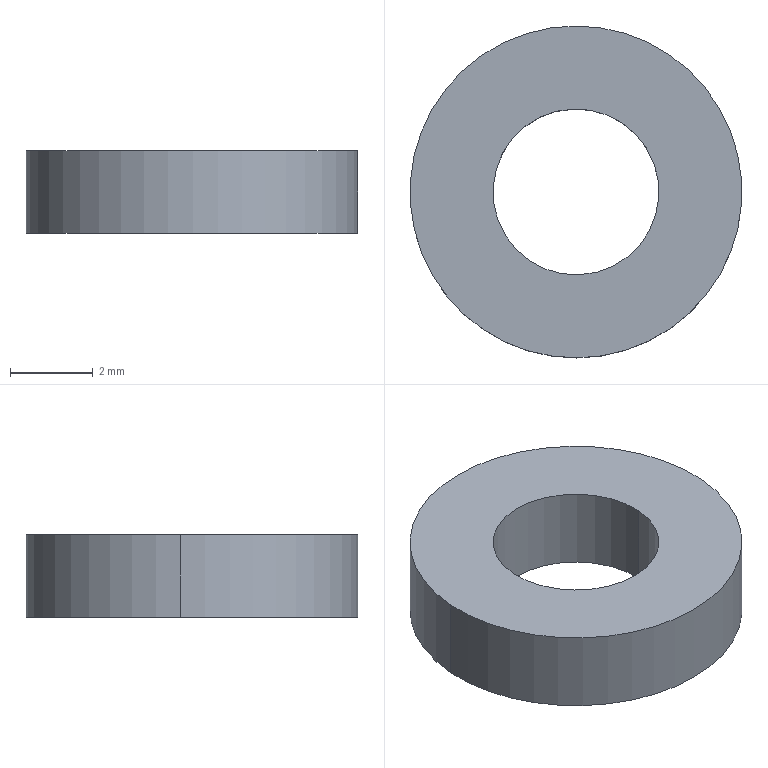Component | SolidWorks | FrontAxisWasher-3 | 1 solid | 6 faces | box 8 x 8 x 2 mm | volume 75 mm3 | cylinder 4 | plane 2 | commonest cylinder face diameters 4 x2 8 x2
build123d program:
from build123d import *

# Parameters (mm, degrees)
SKETCH1_R           = 4
SKETCH1_R_2         = 2
BOSS_EXTRUDE1_DEPTH = 2


with BuildPart() as part:
    # Sketch1 → Boss-Extrude1 (new body)
    with BuildSketch(Plane.XY):
        with Locations((-10, -2.5)):
            Circle(SKETCH1_R)
        with Locations((-10, -2.5)):
            Circle(SKETCH1_R_2, mode=Mode.SUBTRACT)
    extrude(amount=BOSS_EXTRUDE1_DEPTH)


solid = part.part

# Placed as in the assembly
solid = solid.moved(Location((0, 0, -3), (0, 0, 0)))
STEP:
#1=COLOUR_RGB('',0.7922,0.8196,0.9333);
#2=FILL_AREA_STYLE_COLOUR('',#1);
#3=FILL_AREA_STYLE('',(#2));
#4=SURFACE_STYLE_FILL_AREA(#3);
#5=SURFACE_SIDE_STYLE('',(#4));
#6=SURFACE_STYLE_USAGE(.BOTH.,#5);
#7=PRESENTATION_STYLE_ASSIGNMENT((#6));
#8=CARTESIAN_POINT('',(-0.3152,-0.1039,-0.1181));
#9=VERTEX_POINT('',#8);
#10=CARTESIAN_POINT('',(-0.4722,-0.09293,-0.1181));
#11=VERTEX_POINT('',#10);
#12=CARTESIAN_POINT('',(-0.3937,-0.09843,-0.1181));
#13=DIRECTION('',(0.,-0.,-1.));
#14=DIRECTION('',(-0.9976,0.06983,0.));
#15=AXIS2_PLACEMENT_3D('',#12,#13,#14);
#16=CIRCLE('',#15,0.07874);
#17=EDGE_CURVE('',#9,#11,#16,.T.);
#18=ORIENTED_EDGE('',*,*,#17,.T.);
#19=CARTESIAN_POINT('',(-0.4722,-0.09293,-0.03937));
#20=VERTEX_POINT('',#19);
#21=CARTESIAN_POINT('',(-0.4722,-0.09293,-0.1181));
#22=DIRECTION('',(-0.,0.,1.));
#23=VECTOR('',#22,39.37);
#24=LINE('',#21,#23);
#25=EDGE_CURVE('',#11,#20,#24,.T.);
#26=ORIENTED_EDGE('',*,*,#25,.T.);
#27=CARTESIAN_POINT('',(-0.3152,-0.1039,-0.03937));
#28=VERTEX_POINT('',#27);
#29=CARTESIAN_POINT('',(-0.3937,-0.09843,-0.03937));
#30=DIRECTION('',(0.,-0.,-1.));
#31=DIRECTION('',(-0.9976,0.06983,0.));
#32=AXIS2_PLACEMENT_3D('',#29,#30,#31);
#33=CIRCLE('',#32,0.07874);
#34=EDGE_CURVE('',#28,#20,#33,.T.);
#35=ORIENTED_EDGE('',*,*,#34,.F.);
#36=CARTESIAN_POINT('',(-0.3152,-0.1039,-0.1181));
#37=DIRECTION('',(-0.,0.,1.));
#38=VECTOR('',#37,39.37);
#39=LINE('',#36,#38);
#40=EDGE_CURVE('',#9,#28,#39,.T.);
#41=ORIENTED_EDGE('',*,*,#40,.F.);
#42=EDGE_LOOP('',(#18,#26,#35,#41));
#43=FACE_OUTER_BOUND('',#42,.T.);
#44=CARTESIAN_POINT('',(-0.3937,-0.09843,-0.1181));
#45=DIRECTION('',(-0.,0.,1.));
#46=DIRECTION('',(0.9976,-0.06983,0.));
#47=AXIS2_PLACEMENT_3D('',#44,#45,#46);
#48=CYLINDRICAL_SURFACE('',#47,0.07874);
#49=ADVANCED_FACE('',(#43),#48,.F.);
#50=CARTESIAN_POINT('',(-0.5508,-0.08743,-0.1181));
#51=VERTEX_POINT('',#50);
#52=CARTESIAN_POINT('',(-0.2366,-0.1094,-0.1181));
#53=VERTEX_POINT('',#52);
#54=CARTESIAN_POINT('',(-0.3937,-0.09843,-0.1181));
#55=DIRECTION('',(0.,-0.,-1.));
#56=DIRECTION('',(-0.9976,0.06983,0.));
#57=AXIS2_PLACEMENT_3D('',#54,#55,#56);
#58=CIRCLE('',#57,0.1575);
#59=EDGE_CURVE('',#51,#53,#58,.T.);
#60=ORIENTED_EDGE('',*,*,#59,.F.);
#61=CARTESIAN_POINT('',(-0.5508,-0.08743,-0.03937));
#62=VERTEX_POINT('',#61);
#63=CARTESIAN_POINT('',(-0.5508,-0.08743,-0.1181));
#64=DIRECTION('',(-0.,0.,1.));
#65=VECTOR('',#64,39.37);
#66=LINE('',#63,#65);
#67=EDGE_CURVE('',#51,#62,#66,.T.);
#68=ORIENTED_EDGE('',*,*,#67,.T.);
#69=CARTESIAN_POINT('',(-0.2366,-0.1094,-0.03937));
#70=VERTEX_POINT('',#69);
#71=CARTESIAN_POINT('',(-0.3937,-0.09843,-0.03937));
#72=DIRECTION('',(0.,-0.,-1.));
#73=DIRECTION('',(-0.9976,0.06983,0.));
#74=AXIS2_PLACEMENT_3D('',#71,#72,#73);
#75=CIRCLE('',#74,0.1575);
#76=EDGE_CURVE('',#62,#70,#75,.T.);
#77=ORIENTED_EDGE('',*,*,#76,.T.);
#78=CARTESIAN_POINT('',(-0.2366,-0.1094,-0.1181));
#79=DIRECTION('',(-0.,0.,1.));
#80=VECTOR('',#79,39.37);
#81=LINE('',#78,#80);
#82=EDGE_CURVE('',#53,#70,#81,.T.);
#83=ORIENTED_EDGE('',*,*,#82,.F.);
#84=EDGE_LOOP('',(#60,#68,#77,#83));
#85=FACE_OUTER_BOUND('',#84,.T.);
#86=CARTESIAN_POINT('',(-0.3937,-0.09843,-0.1181));
#87=DIRECTION('',(-0.,0.,1.));
#88=DIRECTION('',(0.9976,-0.06983,0.));
#89=AXIS2_PLACEMENT_3D('',#86,#87,#88);
#90=CYLINDRICAL_SURFACE('',#89,0.1575);
#91=ADVANCED_FACE('',(#85),#90,.T.);
#92=CARTESIAN_POINT('',(-0.3937,-0.09843,-0.1181));
#93=DIRECTION('',(0.,-0.,-1.));
#94=DIRECTION('',(-0.9976,0.06983,0.));
#95=AXIS2_PLACEMENT_3D('',#92,#93,#94);
#96=CIRCLE('',#95,0.1575);
#97=EDGE_CURVE('',#53,#51,#96,.T.);
#98=ORIENTED_EDGE('',*,*,#97,.T.);
#99=ORIENTED_EDGE('',*,*,#59,.T.);
#100=EDGE_LOOP('',(#98,#99));
#101=FACE_OUTER_BOUND('',#100,.T.);
#102=ORIENTED_EDGE('',*,*,#17,.F.);
#103=CARTESIAN_POINT('',(-0.3937,-0.09843,-0.1181));
#104=DIRECTION('',(0.,-0.,-1.));
#105=DIRECTION('',(-0.9976,0.06983,0.));
#106=AXIS2_PLACEMENT_3D('',#103,#104,#105);
#107=CIRCLE('',#106,0.07874);
#108=EDGE_CURVE('',#11,#9,#107,.T.);
#109=ORIENTED_EDGE('',*,*,#108,.F.);
#110=EDGE_LOOP('',(#102,#109));
#111=FACE_BOUND('',#110,.T.);
#112=CARTESIAN_POINT('',(-0.3937,-0.09843,-0.1181));
#113=DIRECTION('',(-0.,-0.,-1.));
#114=DIRECTION('',(-0.9976,0.06983,0.));
#115=AXIS2_PLACEMENT_3D('',#112,#113,#114);
#116=PLANE('',#115);
#117=ADVANCED_FACE('',(#101,#111),#116,.T.);
#118=CARTESIAN_POINT('',(-0.3937,-0.09843,-0.03937));
#119=DIRECTION('',(0.,-0.,-1.));
#120=DIRECTION('',(-0.9976,0.06983,0.));
#121=AXIS2_PLACEMENT_3D('',#118,#119,#120);
#122=CIRCLE('',#121,0.1575);
#123=EDGE_CURVE('',#70,#62,#122,.T.);
#124=ORIENTED_EDGE('',*,*,#123,.F.);
#125=ORIENTED_EDGE('',*,*,#76,.F.);
#126=EDGE_LOOP('',(#124,#125));
#127=FACE_OUTER_BOUND('',#126,.T.);
#128=ORIENTED_EDGE('',*,*,#34,.T.);
#129=CARTESIAN_POINT('',(-0.3937,-0.09843,-0.03937));
#130=DIRECTION('',(0.,-0.,-1.));
#131=DIRECTION('',(-0.9976,0.06983,0.));
#132=AXIS2_PLACEMENT_3D('',#129,#130,#131);
#133=CIRCLE('',#132,0.07874);
#134=EDGE_CURVE('',#20,#28,#133,.T.);
#135=ORIENTED_EDGE('',*,*,#134,.T.);
#136=EDGE_LOOP('',(#128,#135));
#137=FACE_BOUND('',#136,.T.);
#138=CARTESIAN_POINT('',(-0.3937,-0.09843,-0.03937));
#139=DIRECTION('',(-0.,-0.,-1.));
#140=DIRECTION('',(-0.9976,0.06983,0.));
#141=AXIS2_PLACEMENT_3D('',#138,#139,#140);
#142=PLANE('',#141);
#143=ADVANCED_FACE('',(#127,#137),#142,.F.);
#144=ORIENTED_EDGE('',*,*,#67,.F.);
#145=ORIENTED_EDGE('',*,*,#97,.F.);
#146=ORIENTED_EDGE('',*,*,#82,.T.);
#147=ORIENTED_EDGE('',*,*,#123,.T.);
#148=EDGE_LOOP('',(#144,#145,#146,#147));
#149=FACE_OUTER_BOUND('',#148,.T.);
#150=CARTESIAN_POINT('',(-0.3937,-0.09843,-0.1181));
#151=DIRECTION('',(-0.,0.,1.));
#152=DIRECTION('',(0.9976,-0.06983,0.));
#153=AXIS2_PLACEMENT_3D('',#150,#151,#152);
#154=CYLINDRICAL_SURFACE('',#153,0.1575);
#155=ADVANCED_FACE('',(#149),#154,.T.);
#156=ORIENTED_EDGE('',*,*,#25,.F.);
#157=ORIENTED_EDGE('',*,*,#108,.T.);
#158=ORIENTED_EDGE('',*,*,#40,.T.);
#159=ORIENTED_EDGE('',*,*,#134,.F.);
#160=EDGE_LOOP('',(#156,#157,#158,#159));
#161=FACE_OUTER_BOUND('',#160,.T.);
#162=CARTESIAN_POINT('',(-0.3937,-0.09843,-0.1181));
#163=DIRECTION('',(-0.,0.,1.));
#164=DIRECTION('',(0.9976,-0.06983,0.));
#165=AXIS2_PLACEMENT_3D('',#162,#163,#164);
#166=CYLINDRICAL_SURFACE('',#165,0.07874);
#167=ADVANCED_FACE('',(#161),#166,.F.);
#168=CLOSED_SHELL('',(#49,#91,#117,#143,#155,#167));
#169=MANIFOLD_SOLID_BREP('',#168);
#170=STYLED_ITEM('',(#7),#169);
#171=PRESENTATION_LAYER_ASSIGNMENT('','',(#170));
#172=(LENGTH_UNIT()NAMED_UNIT(*)SI_UNIT($,.METRE.));
#173=LENGTH_MEASURE_WITH_UNIT(LENGTH_MEASURE(0.0254),#172);
#174=DIMENSIONAL_EXPONENTS(1.,0.,0.,0.,0.,0.,0.);
#175=(CONVERSION_BASED_UNIT('',#173)LENGTH_UNIT()NAMED_UNIT(#174));
#176=UNCERTAINTY_MEASURE_WITH_UNIT(LENGTH_MEASURE(0.00001),#175,'','');
#177=(NAMED_UNIT(*)PLANE_ANGLE_UNIT()SI_UNIT($,.RADIAN.));
#178=(NAMED_UNIT(*)SI_UNIT($,.STERADIAN.)SOLID_ANGLE_UNIT());
#179=(GEOMETRIC_REPRESENTATION_CONTEXT(3)GLOBAL_UNCERTAINTY_ASSIGNED_CONTEXT((#176))GLOBAL_UNIT_ASSIGNED_CONTEXT((#175,#177,#178))REPRESENTATION_CONTEXT('',''));
#180=MECHANICAL_DESIGN_GEOMETRIC_PRESENTATION_REPRESENTATION('',(#170),#179);
#181=CARTESIAN_POINT('',(0.,0.,0.));
#182=DIRECTION('',(0.,0.,1.));
#183=DIRECTION('',(1.,0.,0.));
#184=AXIS2_PLACEMENT_3D('',#181,#182,#183);
#185=(LENGTH_UNIT()NAMED_UNIT(*)SI_UNIT($,.METRE.));
#186=LENGTH_MEASURE_WITH_UNIT(LENGTH_MEASURE(0.0254),#185);
#187=DIMENSIONAL_EXPONENTS(1.,0.,0.,0.,0.,0.,0.);
#188=(CONVERSION_BASED_UNIT('',#186)LENGTH_UNIT()NAMED_UNIT(#187));
#189=UNCERTAINTY_MEASURE_WITH_UNIT(LENGTH_MEASURE(0.00001),#188,'','');
#190=(NAMED_UNIT(*)PLANE_ANGLE_UNIT()SI_UNIT($,.RADIAN.));
#191=(NAMED_UNIT(*)SI_UNIT($,.STERADIAN.)SOLID_ANGLE_UNIT());
#192=(GEOMETRIC_REPRESENTATION_CONTEXT(3)GLOBAL_UNCERTAINTY_ASSIGNED_CONTEXT((#189))GLOBAL_UNIT_ASSIGNED_CONTEXT((#188,#190,#191))REPRESENTATION_CONTEXT('',''));
#193=ADVANCED_BREP_SHAPE_REPRESENTATION('',(#169,#184),#192);